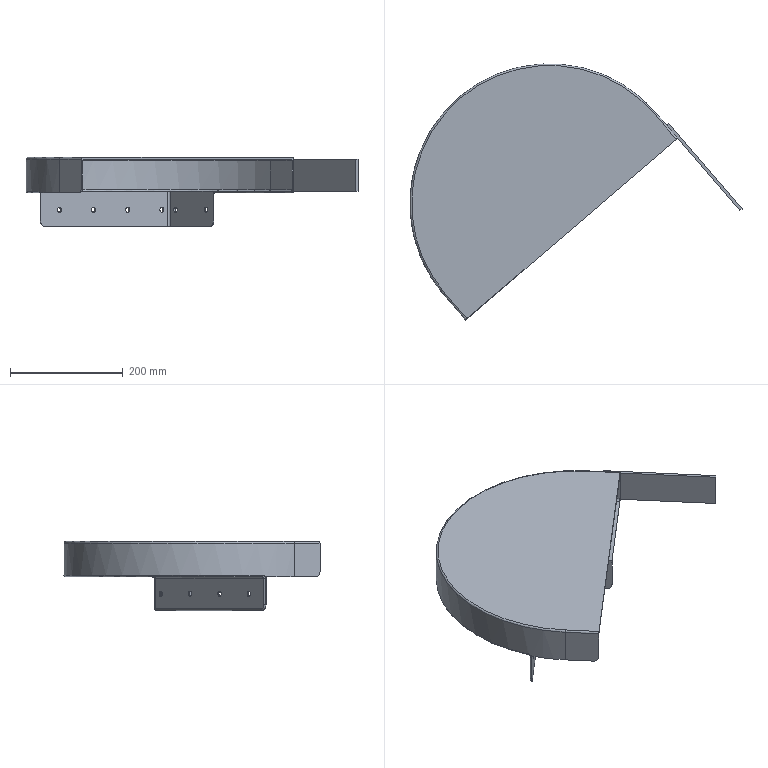Component | SolidWorks | SawBladeGuardB-1 | 2 solids | 62 faces | volume 932659 mm3 | cylinder 30 | plane 21 | torus 8 | spline 3 | commonest cylinder face diameters 6 x14 9.5 x12 490 x1 496 x1 20 x1 12 x1 | material 45